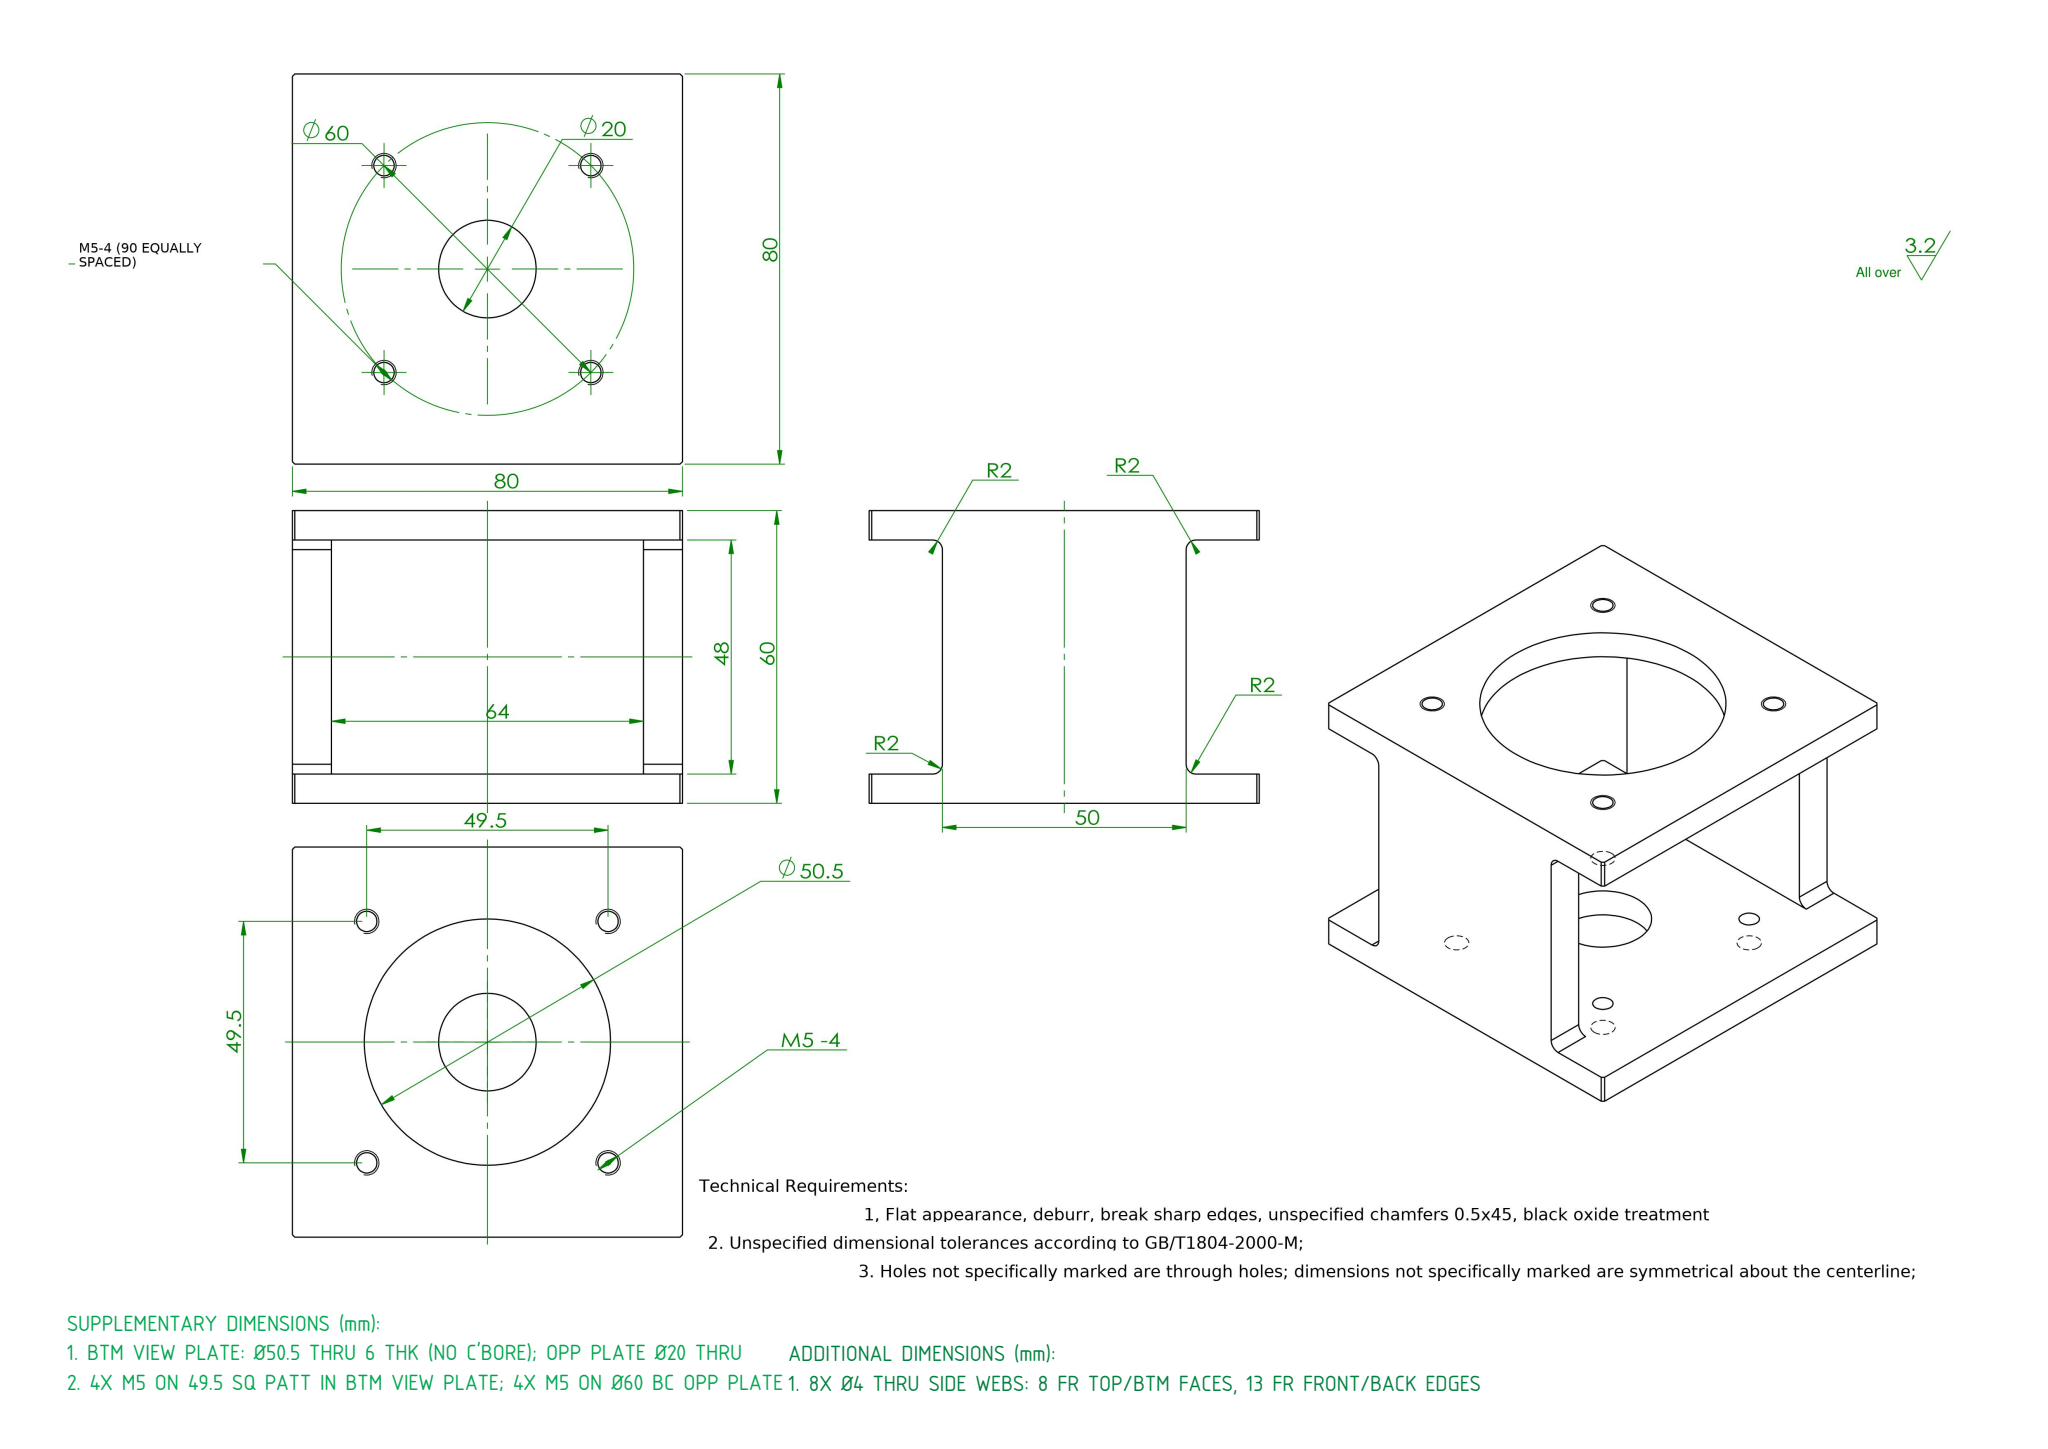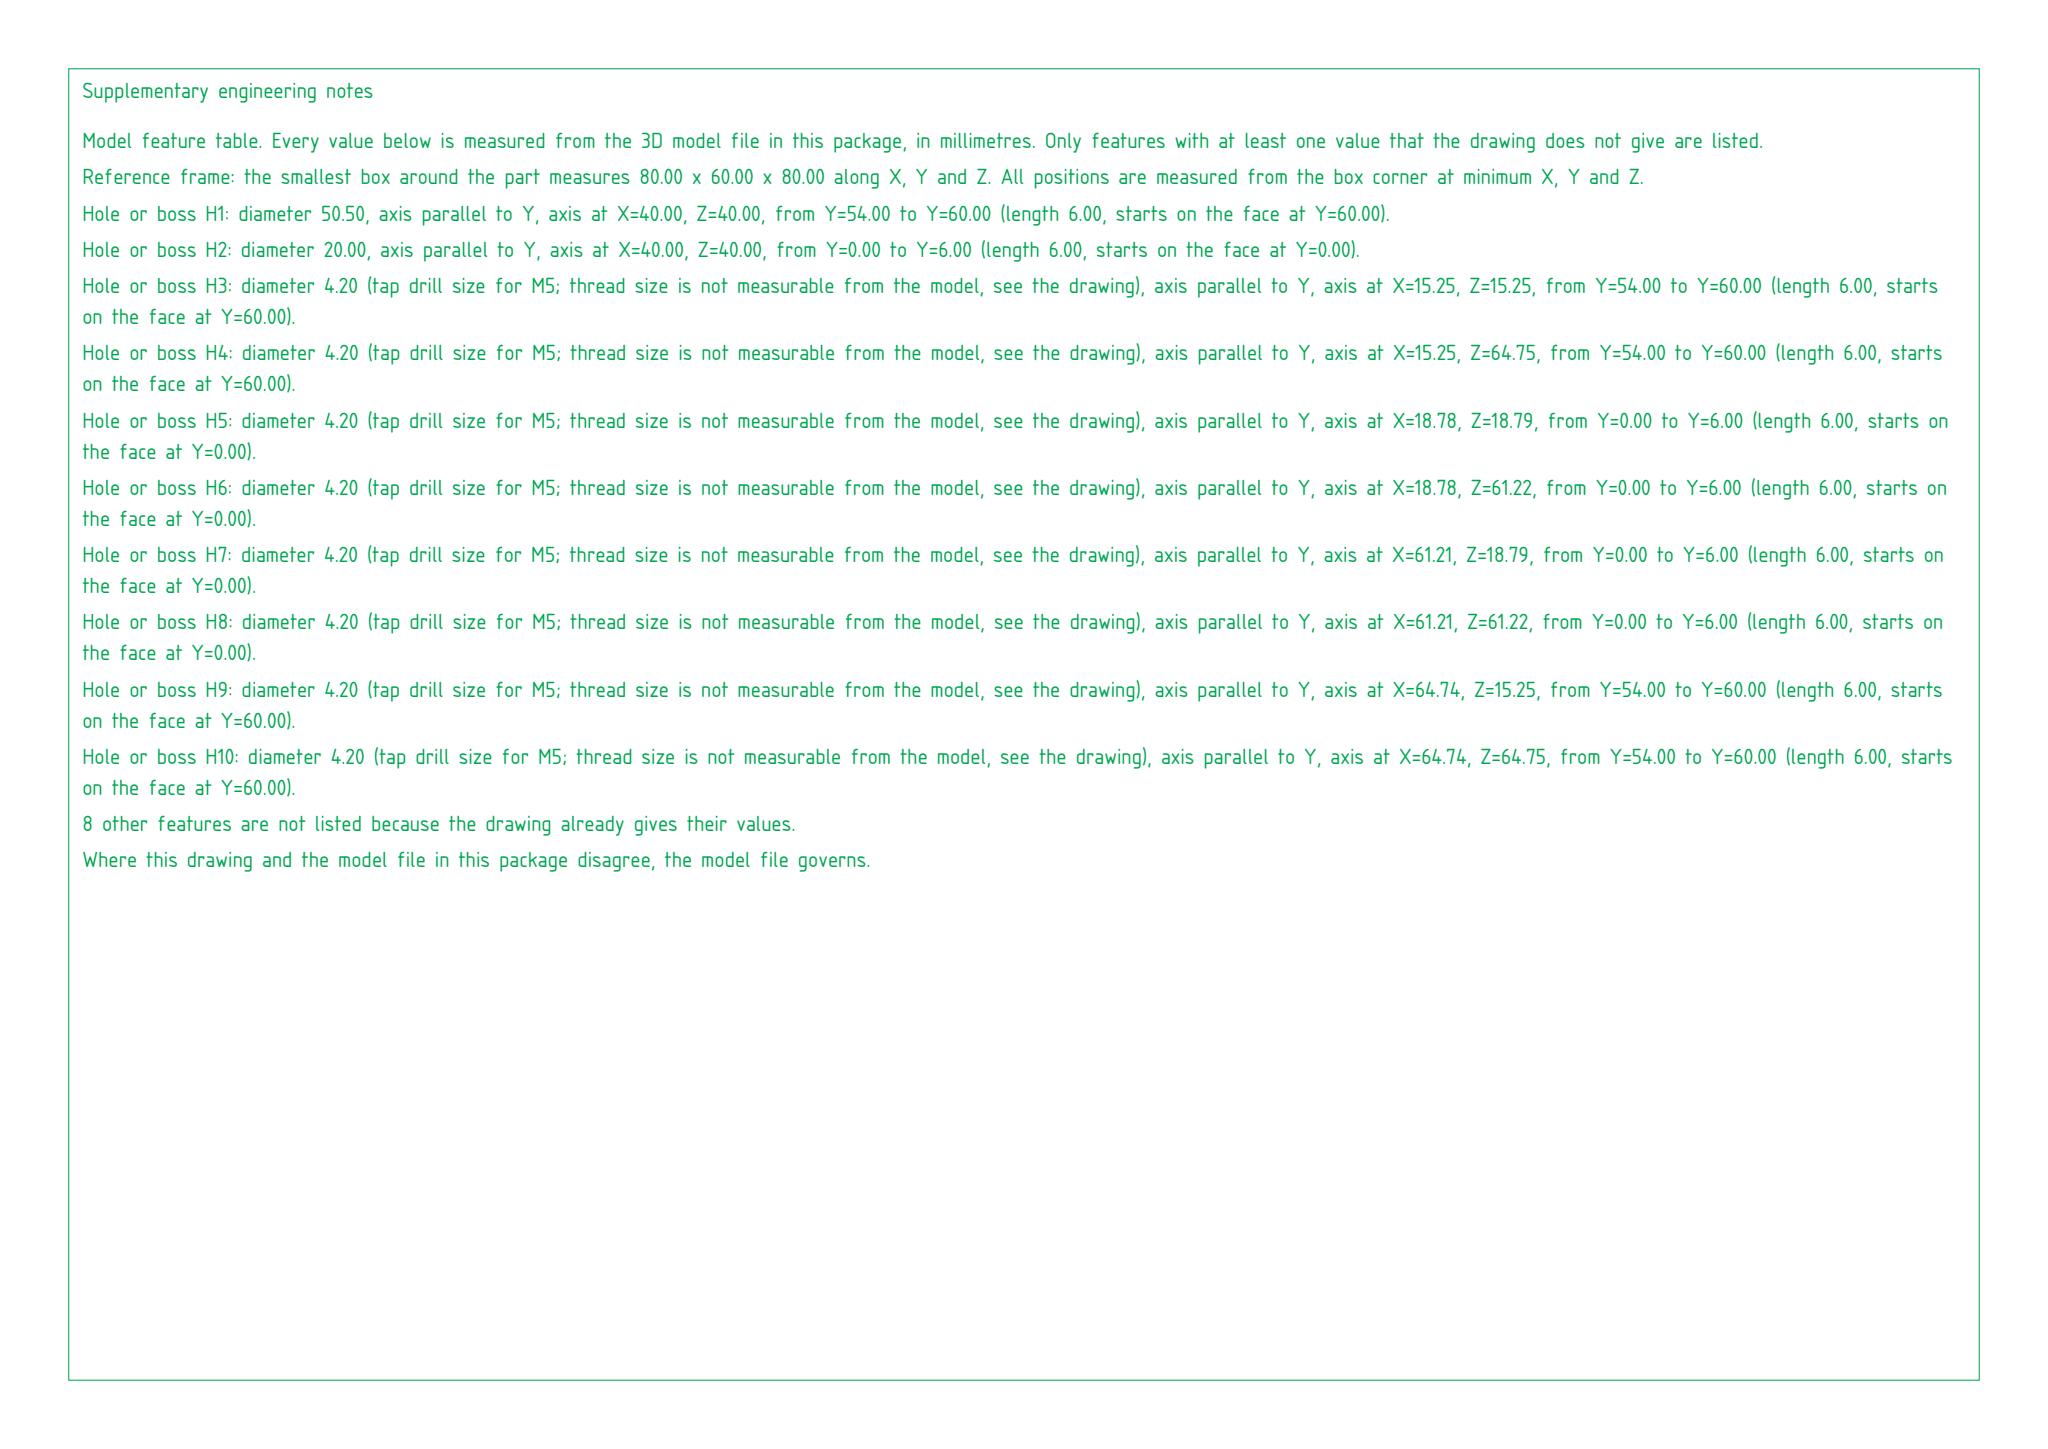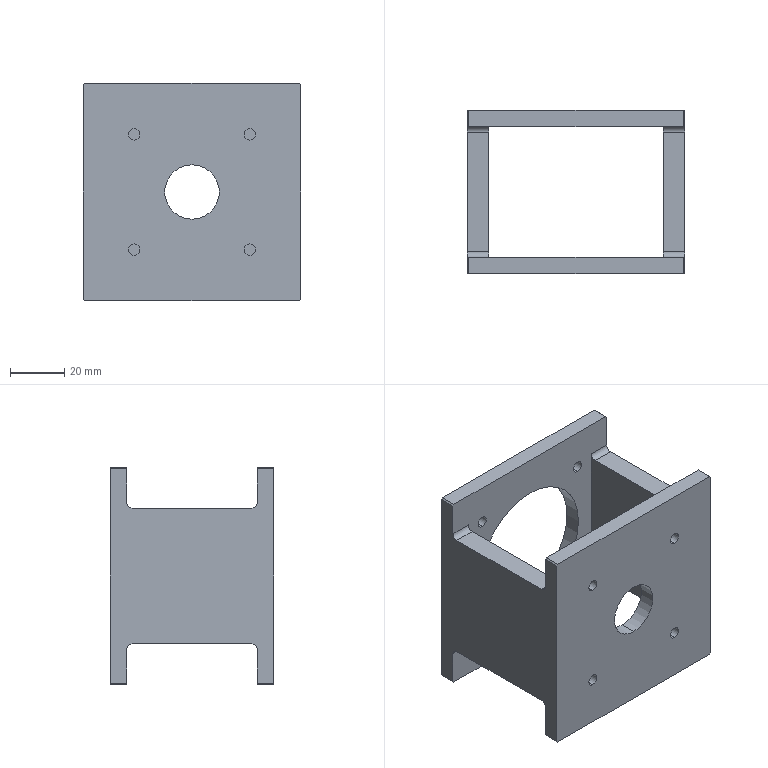Part | SolidWorks | mm | 1 solid | 52 faces | box 80 x 60 x 80 mm | volume 100681 mm3 | cylinder 28 | plane 24 | commonest cylinder face diameters 4.2 x16 4 x8 20 x2 50.5 x2
build123d program:
from build123d import *

# Parameters (mm, degrees)
SKETCH1_W           = 80
SKETCH1_H           = 80
BOSS_EXTRUDE1_DEPTH = 60
SKETCH2_W           = 15
SKETCH2_H           = 48
CUT_EXTRUDE1_DEPTH  = 109.707
SKETCH4_R           = 10
CUT_EXTRUDE3_DEPTH  = 10
CHAMFER2_SIZE       = 0.5
SKETCH5_W           = 64
SKETCH5_H           = 48
CUT_EXTRUDE4_DEPTH  = 60
SKETCH7_R           = 25.25
CUT_EXTRUDE5_DEPTH  = 12
SKETCH10_R          = 10
CUT_EXTRUDE6_DEPTH  = 10
CIRPATTERN1_COUNT   = 4
CIRPATTERN2_COUNT   = 4
FILLET1_R           = 2


with BuildPart() as part:
    # Sketch1 → Boss-Extrude1 (new body)
    with BuildSketch(Plane(origin=(0, 0, 0), x_dir=(1, 0, 0), z_dir=(0, 1, 0))):
        with Locations((-25.964, 2.628)):
            Rectangle(SKETCH1_W, SKETCH1_H)
    extrude(amount=BOSS_EXTRUDE1_DEPTH)

    # Sketch2 → Cut-Extrude1 (cut, through all)
    with BuildSketch(Plane(origin=(14.036, 0, 0), x_dir=(0, 0, -1), z_dir=(1, 0, 0))):
        with Locations((-29.872, 30)):
            Rectangle(SKETCH2_W, SKETCH2_H)
        with Locations((35.128, 30)):
            Rectangle(SKETCH2_W, SKETCH2_H)
    extrude(amount=-CUT_EXTRUDE1_DEPTH, mode=Mode.SUBTRACT)

    # Sketch4 → Cut-Extrude3 (cut)
    with BuildSketch(Plane(origin=(0, 60, 0), x_dir=(1, 0, 0), z_dir=(0, 1, 0))):
        with Locations(Location((-25.964, 2.628, 0), (0, 0, 270))):
            Circle(SKETCH4_R)
    extrude(amount=-CUT_EXTRUDE3_DEPTH, mode=Mode.SUBTRACT)

    # Chamfer2
    chamfer2_edges = [part.edges().sort_by_distance(p)[0] for p in [
        (14.036, 3, 37.372),
        (-65.964, 3, 37.372),
        (-65.964, 3, -42.628),
        (14.036, 3, -42.628),
        (-65.964, 57, -42.628),
        (14.036, 57, -42.628),
        (14.036, 57, 37.372),
        (-65.964, 57, 37.372),
    ]]
    chamfer(chamfer2_edges, length=CHAMFER2_SIZE)

    # Sketch5 → Cut-Extrude4 (cut)
    with BuildSketch(Plane.XY.offset(22.372)):
        with Locations((-25.964, 30)):
            Rectangle(SKETCH5_W, SKETCH5_H)
    extrude(amount=-CUT_EXTRUDE4_DEPTH, mode=Mode.SUBTRACT)

    # Sketch7 → Cut-Extrude5 (cut)
    with BuildSketch(Plane(origin=(0, 60, 0), x_dir=(1, 0, 0), z_dir=(0, 1, 0))):
        with Locations(Location((-25.964, 2.628, 0), (0, 0, 270))):
            Circle(SKETCH7_R)
    extrude(amount=-CUT_EXTRUDE5_DEPTH, mode=Mode.SUBTRACT)

    # Sketch10 → Cut-Extrude6 (cut)
    with BuildSketch(Plane.XZ):
        with Locations(Location((-25.964, -2.628, 0), (0, 0, 270))):
            Circle(SKETCH10_R)
    extrude(amount=-CUT_EXTRUDE6_DEPTH, mode=Mode.SUBTRACT)

    # Sketch8 → M5 Tapped Hole1 (revolve, cut)
    with BuildSketch(Plane(origin=(-47.177, 0, -23.841), x_dir=(0, 0, -1), z_dir=(1, 0, 0))):
        Polygon((0, 0), (0, 13.662), (2.1, 12.4), (2.1, 0), align=None)
    m5_tapped_hole1 = revolve(axis=Axis((-47.177, -6.35, -23.841), (0, 1, 0)), mode=Mode.SUBTRACT)

    # CirPattern1: M5 Tapped Hole1 ×4 about axis
    cirpattern1_axis = Axis((-25.964, 0, -2.628), (0, 1, 0))
    for i in range(1, CIRPATTERN1_COUNT):
        add(m5_tapped_hole1.rotate(cirpattern1_axis, i * 360 / CIRPATTERN1_COUNT), mode=Mode.SUBTRACT)

    # Sketch11 → M5 Tapped Hole2 (revolve, cut)
    with BuildSketch(Plane(origin=(-50.712, 60, 22.121), x_dir=(0, 0, 1), z_dir=(1, 0, 0))):
        Polygon((0, 0), (0, 13.662), (2.1, 12.4), (2.1, 0), align=None)
    m5_tapped_hole2 = revolve(axis=Axis((-50.712, 66.35, 22.121), (0, -1, 0)), mode=Mode.SUBTRACT)

    # CirPattern2: M5 Tapped Hole2 ×4 about axis
    cirpattern2_axis = Axis((-25.964, 0, -2.628), (0, 1, 0))
    for i in range(1, CIRPATTERN2_COUNT):
        add(m5_tapped_hole2.rotate(cirpattern2_axis, i * 360 / CIRPATTERN2_COUNT), mode=Mode.SUBTRACT)

    # Fillet1
    fillet1_edges = [part.edges().sort_by_distance(p)[0] for p in [
        (10.036, 6, -27.628),
        (10.036, 6, 22.372),
        (10.036, 54, 22.372),
        (-61.964, 54, 22.372),
        (-61.964, 6, 22.372),
        (-61.964, 6, -27.628),
        (-61.964, 54, -27.628),
        (10.036, 54, -27.628),
    ]]
    fillet(fillet1_edges, radius=FILLET1_R)


solid = part.part